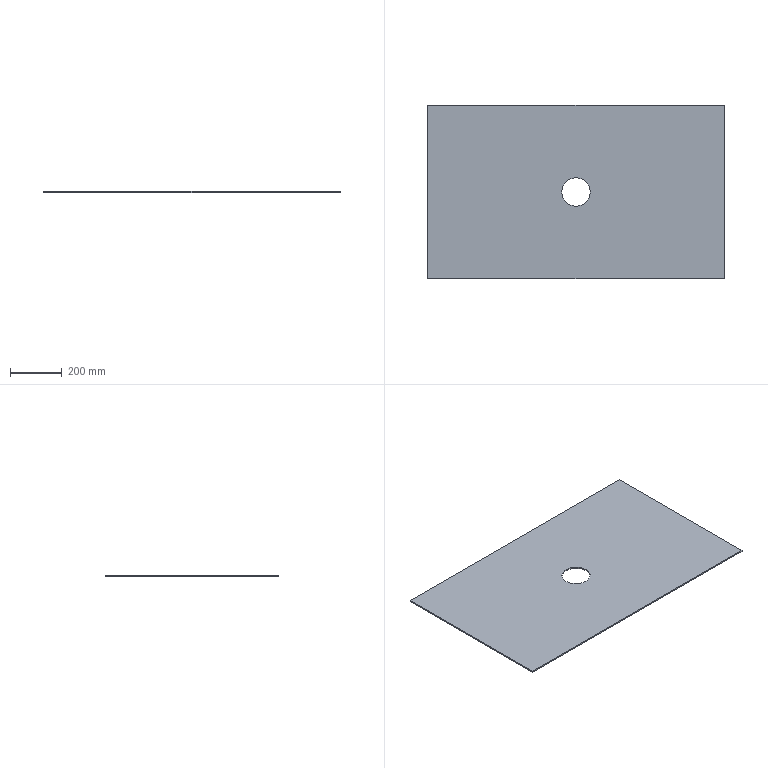Component | SolidWorks | TopCoverPlate-1 | 1 solid | 8 faces | box 1145 x 670 x 5 mm | volume 3788233 mm3 | plane 6 | cylinder 2 | commonest cylinder face diameters 110 x2
build123d program:
from build123d import *

# Parameters (mm, degrees)
SKETCH1_W           = 1145
SKETCH1_H           = 670
BOSS_EXTRUDE1_DEPTH = 5
SKETCH2_R           = 55
CUT_EXTRUDE1_DEPTH  = 80


with BuildPart() as part:
    # Sketch1 → Boss-Extrude1 (new body)
    with BuildSketch(Plane.XY):
        with Locations((572.5, -335)):
            Rectangle(SKETCH1_W, SKETCH1_H)
    extrude(amount=BOSS_EXTRUDE1_DEPTH)

    # Sketch2 → Cut-Extrude1 (cut)
    with BuildSketch(Plane.XY.offset(5)):
        with Locations((572.5, -335)):
            Circle(SKETCH2_R)
    extrude(amount=-CUT_EXTRUDE1_DEPTH, mode=Mode.SUBTRACT)


solid = part.part

# Placed as in the assembly
solid = solid.moved(Location((-28.047, 652.523, 450), (0, 0, 0)))
STEP:
#1=COLOUR_RGB('',0.7922,0.8196,0.9333);
#2=FILL_AREA_STYLE_COLOUR('',#1);
#3=FILL_AREA_STYLE('',(#2));
#4=SURFACE_STYLE_FILL_AREA(#3);
#5=SURFACE_SIDE_STYLE('',(#4));
#6=SURFACE_STYLE_USAGE(.BOTH.,#5);
#7=PRESENTATION_STYLE_ASSIGNMENT((#6));
#8=CARTESIAN_POINT('',(19.27,12.501,17.717));
#9=VERTEX_POINT('',#8);
#10=CARTESIAN_POINT('',(23.601,12.501,17.717));
#11=VERTEX_POINT('',#10);
#12=CARTESIAN_POINT('',(21.435,12.501,17.717));
#13=DIRECTION('',(0.,0.,1.));
#14=DIRECTION('',(1.,0.,0.));
#15=AXIS2_PLACEMENT_3D('',#12,#13,#14);
#16=CIRCLE('',#15,2.165);
#17=EDGE_CURVE('',#9,#11,#16,.T.);
#18=ORIENTED_EDGE('',*,*,#17,.F.);
#19=CARTESIAN_POINT('',(19.27,12.501,17.913));
#20=VERTEX_POINT('',#19);
#21=CARTESIAN_POINT('',(19.27,12.501,14.764));
#22=DIRECTION('',(0.,0.,1.));
#23=VECTOR('',#22,39.37);
#24=LINE('',#21,#23);
#25=EDGE_CURVE('',#9,#20,#24,.T.);
#26=ORIENTED_EDGE('',*,*,#25,.T.);
#27=CARTESIAN_POINT('',(23.601,12.501,17.913));
#28=VERTEX_POINT('',#27);
#29=CARTESIAN_POINT('',(21.435,12.501,17.913));
#30=DIRECTION('',(0.,0.,1.));
#31=DIRECTION('',(1.,0.,0.));
#32=AXIS2_PLACEMENT_3D('',#29,#30,#31);
#33=CIRCLE('',#32,2.165);
#34=EDGE_CURVE('',#20,#28,#33,.T.);
#35=ORIENTED_EDGE('',*,*,#34,.T.);
#36=CARTESIAN_POINT('',(23.601,12.501,14.764));
#37=DIRECTION('',(0.,0.,1.));
#38=VECTOR('',#37,39.37);
#39=LINE('',#36,#38);
#40=EDGE_CURVE('',#11,#28,#39,.T.);
#41=ORIENTED_EDGE('',*,*,#40,.F.);
#42=EDGE_LOOP('',(#18,#26,#35,#41));
#43=FACE_OUTER_BOUND('',#42,.T.);
#44=CARTESIAN_POINT('',(21.435,12.501,14.764));
#45=DIRECTION('',(0.,0.,1.));
#46=DIRECTION('',(1.,0.,0.));
#47=AXIS2_PLACEMENT_3D('',#44,#45,#46);
#48=CYLINDRICAL_SURFACE('',#47,2.165);
#49=ADVANCED_FACE('',(#43),#48,.F.);
#50=CARTESIAN_POINT('',(-1.104,25.69,17.717));
#51=VERTEX_POINT('',#50);
#52=CARTESIAN_POINT('',(-1.104,-0.6881,17.717));
#53=VERTEX_POINT('',#52);
#54=CARTESIAN_POINT('',(-1.104,25.69,17.717));
#55=DIRECTION('',(0.,-1.,0.));
#56=VECTOR('',#55,39.37);
#57=LINE('',#54,#56);
#58=EDGE_CURVE('',#51,#53,#57,.T.);
#59=ORIENTED_EDGE('',*,*,#58,.T.);
#60=CARTESIAN_POINT('',(-1.104,-0.6881,17.913));
#61=VERTEX_POINT('',#60);
#62=CARTESIAN_POINT('',(-1.104,-0.6881,17.913));
#63=DIRECTION('',(0.,0.,-1.));
#64=VECTOR('',#63,39.37);
#65=LINE('',#62,#64);
#66=EDGE_CURVE('',#61,#53,#65,.T.);
#67=ORIENTED_EDGE('',*,*,#66,.F.);
#68=CARTESIAN_POINT('',(-1.104,25.69,17.913));
#69=VERTEX_POINT('',#68);
#70=CARTESIAN_POINT('',(-1.104,25.69,17.913));
#71=DIRECTION('',(0.,-1.,0.));
#72=VECTOR('',#71,39.37);
#73=LINE('',#70,#72);
#74=EDGE_CURVE('',#69,#61,#73,.T.);
#75=ORIENTED_EDGE('',*,*,#74,.F.);
#76=CARTESIAN_POINT('',(-1.104,25.69,17.913));
#77=DIRECTION('',(0.,0.,-1.));
#78=VECTOR('',#77,39.37);
#79=LINE('',#76,#78);
#80=EDGE_CURVE('',#69,#51,#79,.T.);
#81=ORIENTED_EDGE('',*,*,#80,.T.);
#82=EDGE_LOOP('',(#59,#67,#75,#81));
#83=FACE_OUTER_BOUND('',#82,.T.);
#84=CARTESIAN_POINT('',(-1.104,25.69,17.913));
#85=DIRECTION('',(1.,0.,0.));
#86=DIRECTION('',(-0.,1.,0.));
#87=AXIS2_PLACEMENT_3D('',#84,#85,#86);
#88=PLANE('',#87);
#89=ADVANCED_FACE('',(#83),#88,.F.);
#90=CARTESIAN_POINT('',(43.975,-0.6881,17.717));
#91=VERTEX_POINT('',#90);
#92=CARTESIAN_POINT('',(-1.104,-0.6881,17.717));
#93=DIRECTION('',(1.,0.,0.));
#94=VECTOR('',#93,39.37);
#95=LINE('',#92,#94);
#96=EDGE_CURVE('',#53,#91,#95,.T.);
#97=ORIENTED_EDGE('',*,*,#96,.T.);
#98=CARTESIAN_POINT('',(43.975,-0.6881,17.913));
#99=VERTEX_POINT('',#98);
#100=CARTESIAN_POINT('',(43.975,-0.6881,17.913));
#101=DIRECTION('',(0.,0.,-1.));
#102=VECTOR('',#101,39.37);
#103=LINE('',#100,#102);
#104=EDGE_CURVE('',#99,#91,#103,.T.);
#105=ORIENTED_EDGE('',*,*,#104,.F.);
#106=CARTESIAN_POINT('',(-1.104,-0.6881,17.913));
#107=DIRECTION('',(1.,0.,0.));
#108=VECTOR('',#107,39.37);
#109=LINE('',#106,#108);
#110=EDGE_CURVE('',#61,#99,#109,.T.);
#111=ORIENTED_EDGE('',*,*,#110,.F.);
#112=ORIENTED_EDGE('',*,*,#66,.T.);
#113=EDGE_LOOP('',(#97,#105,#111,#112));
#114=FACE_OUTER_BOUND('',#113,.T.);
#115=CARTESIAN_POINT('',(-1.104,-0.6881,17.913));
#116=DIRECTION('',(0.,1.,0.));
#117=DIRECTION('',(0.,0.,1.));
#118=AXIS2_PLACEMENT_3D('',#115,#116,#117);
#119=PLANE('',#118);
#120=ADVANCED_FACE('',(#114),#119,.F.);
#121=CARTESIAN_POINT('',(43.975,25.69,17.717));
#122=VERTEX_POINT('',#121);
#123=CARTESIAN_POINT('',(43.975,25.69,17.717));
#124=DIRECTION('',(0.,1.,0.));
#125=VECTOR('',#124,39.37);
#126=LINE('',#123,#125);
#127=EDGE_CURVE('',#91,#122,#126,.T.);
#128=ORIENTED_EDGE('',*,*,#127,.T.);
#129=CARTESIAN_POINT('',(43.975,25.69,17.913));
#130=VERTEX_POINT('',#129);
#131=CARTESIAN_POINT('',(43.975,25.69,17.913));
#132=DIRECTION('',(0.,0.,-1.));
#133=VECTOR('',#132,39.37);
#134=LINE('',#131,#133);
#135=EDGE_CURVE('',#130,#122,#134,.T.);
#136=ORIENTED_EDGE('',*,*,#135,.F.);
#137=CARTESIAN_POINT('',(43.975,25.69,17.913));
#138=DIRECTION('',(0.,1.,0.));
#139=VECTOR('',#138,39.37);
#140=LINE('',#137,#139);
#141=EDGE_CURVE('',#99,#130,#140,.T.);
#142=ORIENTED_EDGE('',*,*,#141,.F.);
#143=ORIENTED_EDGE('',*,*,#104,.T.);
#144=EDGE_LOOP('',(#128,#136,#142,#143));
#145=FACE_OUTER_BOUND('',#144,.T.);
#146=CARTESIAN_POINT('',(43.975,25.69,17.913));
#147=DIRECTION('',(-1.,0.,0.));
#148=DIRECTION('',(0.,0.,1.));
#149=AXIS2_PLACEMENT_3D('',#146,#147,#148);
#150=PLANE('',#149);
#151=ADVANCED_FACE('',(#145),#150,.F.);
#152=CARTESIAN_POINT('',(-1.104,25.69,17.717));
#153=DIRECTION('',(-1.,0.,0.));
#154=VECTOR('',#153,39.37);
#155=LINE('',#152,#154);
#156=EDGE_CURVE('',#122,#51,#155,.T.);
#157=ORIENTED_EDGE('',*,*,#156,.T.);
#158=ORIENTED_EDGE('',*,*,#80,.F.);
#159=CARTESIAN_POINT('',(-1.104,25.69,17.913));
#160=DIRECTION('',(-1.,0.,0.));
#161=VECTOR('',#160,39.37);
#162=LINE('',#159,#161);
#163=EDGE_CURVE('',#130,#69,#162,.T.);
#164=ORIENTED_EDGE('',*,*,#163,.F.);
#165=ORIENTED_EDGE('',*,*,#135,.T.);
#166=EDGE_LOOP('',(#157,#158,#164,#165));
#167=FACE_OUTER_BOUND('',#166,.T.);
#168=CARTESIAN_POINT('',(-1.104,25.69,17.913));
#169=DIRECTION('',(0.,-1.,0.));
#170=DIRECTION('',(0.,0.,-1.));
#171=AXIS2_PLACEMENT_3D('',#168,#169,#170);
#172=PLANE('',#171);
#173=ADVANCED_FACE('',(#167),#172,.F.);
#174=CARTESIAN_POINT('',(21.435,12.501,17.913));
#175=DIRECTION('',(0.,0.,1.));
#176=DIRECTION('',(1.,0.,0.));
#177=AXIS2_PLACEMENT_3D('',#174,#175,#176);
#178=CIRCLE('',#177,2.165);
#179=EDGE_CURVE('',#28,#20,#178,.T.);
#180=ORIENTED_EDGE('',*,*,#179,.F.);
#181=ORIENTED_EDGE('',*,*,#34,.F.);
#182=EDGE_LOOP('',(#180,#181));
#183=FACE_BOUND('',#182,.T.);
#184=ORIENTED_EDGE('',*,*,#74,.T.);
#185=ORIENTED_EDGE('',*,*,#110,.T.);
#186=ORIENTED_EDGE('',*,*,#141,.T.);
#187=ORIENTED_EDGE('',*,*,#163,.T.);
#188=EDGE_LOOP('',(#184,#185,#186,#187));
#189=FACE_OUTER_BOUND('',#188,.T.);
#190=CARTESIAN_POINT('',(-1.104,25.69,17.913));
#191=DIRECTION('',(0.,0.,1.));
#192=DIRECTION('',(1.,0.,0.));
#193=AXIS2_PLACEMENT_3D('',#190,#191,#192);
#194=PLANE('',#193);
#195=ADVANCED_FACE('',(#183,#189),#194,.T.);
#196=CARTESIAN_POINT('',(21.435,12.501,17.717));
#197=DIRECTION('',(0.,0.,1.));
#198=DIRECTION('',(1.,0.,0.));
#199=AXIS2_PLACEMENT_3D('',#196,#197,#198);
#200=CIRCLE('',#199,2.165);
#201=EDGE_CURVE('',#11,#9,#200,.T.);
#202=ORIENTED_EDGE('',*,*,#201,.T.);
#203=ORIENTED_EDGE('',*,*,#17,.T.);
#204=EDGE_LOOP('',(#202,#203));
#205=FACE_BOUND('',#204,.T.);
#206=ORIENTED_EDGE('',*,*,#58,.F.);
#207=ORIENTED_EDGE('',*,*,#156,.F.);
#208=ORIENTED_EDGE('',*,*,#127,.F.);
#209=ORIENTED_EDGE('',*,*,#96,.F.);
#210=EDGE_LOOP('',(#206,#207,#208,#209));
#211=FACE_OUTER_BOUND('',#210,.T.);
#212=CARTESIAN_POINT('',(-1.104,25.69,17.717));
#213=DIRECTION('',(0.,0.,1.));
#214=DIRECTION('',(1.,0.,0.));
#215=AXIS2_PLACEMENT_3D('',#212,#213,#214);
#216=PLANE('',#215);
#217=ADVANCED_FACE('',(#205,#211),#216,.F.);
#218=ORIENTED_EDGE('',*,*,#25,.F.);
#219=ORIENTED_EDGE('',*,*,#201,.F.);
#220=ORIENTED_EDGE('',*,*,#40,.T.);
#221=ORIENTED_EDGE('',*,*,#179,.T.);
#222=EDGE_LOOP('',(#218,#219,#220,#221));
#223=FACE_OUTER_BOUND('',#222,.T.);
#224=CARTESIAN_POINT('',(21.435,12.501,14.764));
#225=DIRECTION('',(0.,0.,1.));
#226=DIRECTION('',(1.,0.,0.));
#227=AXIS2_PLACEMENT_3D('',#224,#225,#226);
#228=CYLINDRICAL_SURFACE('',#227,2.165);
#229=ADVANCED_FACE('',(#223),#228,.F.);
#230=CLOSED_SHELL('',(#49,#89,#120,#151,#173,#195,#217,#229));
#231=MANIFOLD_SOLID_BREP('',#230);
#232=STYLED_ITEM('',(#7),#231);
#233=PRESENTATION_LAYER_ASSIGNMENT('','',(#232));
#234=(LENGTH_UNIT()NAMED_UNIT(*)SI_UNIT($,.METRE.));
#235=LENGTH_MEASURE_WITH_UNIT(LENGTH_MEASURE(0.0254),#234);
#236=DIMENSIONAL_EXPONENTS(1.,0.,0.,0.,0.,0.,0.);
#237=(CONVERSION_BASED_UNIT('',#235)LENGTH_UNIT()NAMED_UNIT(#236));
#238=UNCERTAINTY_MEASURE_WITH_UNIT(LENGTH_MEASURE(0.00001),#237,'','');
#239=(NAMED_UNIT(*)PLANE_ANGLE_UNIT()SI_UNIT($,.RADIAN.));
#240=(NAMED_UNIT(*)SI_UNIT($,.STERADIAN.)SOLID_ANGLE_UNIT());
#241=(GEOMETRIC_REPRESENTATION_CONTEXT(3)GLOBAL_UNCERTAINTY_ASSIGNED_CONTEXT((#238))GLOBAL_UNIT_ASSIGNED_CONTEXT((#237,#239,#240))REPRESENTATION_CONTEXT('',''));
#242=MECHANICAL_DESIGN_GEOMETRIC_PRESENTATION_REPRESENTATION('',(#232),#241);
#243=CARTESIAN_POINT('',(0.,0.,0.));
#244=DIRECTION('',(0.,0.,1.));
#245=DIRECTION('',(1.,0.,0.));
#246=AXIS2_PLACEMENT_3D('',#243,#244,#245);
#247=(LENGTH_UNIT()NAMED_UNIT(*)SI_UNIT($,.METRE.));
#248=LENGTH_MEASURE_WITH_UNIT(LENGTH_MEASURE(0.0254),#247);
#249=DIMENSIONAL_EXPONENTS(1.,0.,0.,0.,0.,0.,0.);
#250=(CONVERSION_BASED_UNIT('',#248)LENGTH_UNIT()NAMED_UNIT(#249));
#251=UNCERTAINTY_MEASURE_WITH_UNIT(LENGTH_MEASURE(0.00001),#250,'','');
#252=(NAMED_UNIT(*)PLANE_ANGLE_UNIT()SI_UNIT($,.RADIAN.));
#253=(NAMED_UNIT(*)SI_UNIT($,.STERADIAN.)SOLID_ANGLE_UNIT());
#254=(GEOMETRIC_REPRESENTATION_CONTEXT(3)GLOBAL_UNCERTAINTY_ASSIGNED_CONTEXT((#251))GLOBAL_UNIT_ASSIGNED_CONTEXT((#250,#252,#253))REPRESENTATION_CONTEXT('',''));
#255=ADVANCED_BREP_SHAPE_REPRESENTATION('',(#231,#246),#254);